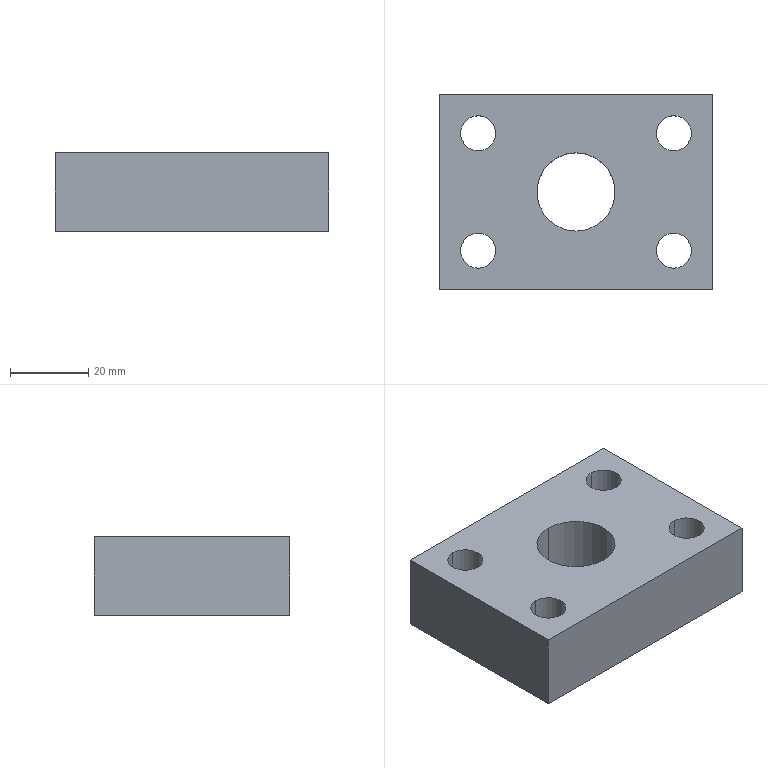Component | SolidWorks | UpperSideBeltXG-XG1-1_AdjustingNutXG1-1 | 1 solid | 16 faces | box 70 x 50 x 20 mm | volume 58627 mm3 | cylinder 10 | plane 6 | commonest cylinder face diameters 9 x8 20 x2
build123d program:
from build123d import *

# Parameters (mm, degrees)
SKETCH1_W                = 70
SKETCH1_H                = 50
BOSS_EXTRUDE1_DEPTH      = 10
F_9_0_9_DIAMETER_HOLE1_D = 9
M20_TAPPED_HOLE1_D       = 20


with BuildPart() as part:
    # Sketch1 → Boss-Extrude1 (new, symmetric)
    with BuildSketch(Plane(origin=(0, 0, 0), x_dir=(1, 0, 0), z_dir=(0, 1, 0))):
        Rectangle(SKETCH1_W, SKETCH1_H)
    extrude(amount=BOSS_EXTRUDE1_DEPTH, both=True)

    # 9.0 _9_ Diameter Hole1 (through all)
    with Locations(Plane(origin=(0, 10, 0), x_dir=(1, 0, 0), z_dir=(0, 1, 0))):
        with Locations((-25, 15), (-25, -15), (25, 15), (25, -15)):
            Hole(F_9_0_9_DIAMETER_HOLE1_D / 2)

    # M20 Tapped Hole1 (through all)
    with Locations(Plane(origin=(0, 10, 0), x_dir=(1, 0, 0), z_dir=(0, 1, 0))):
        with Locations((0, 0)):
            Hole(M20_TAPPED_HOLE1_D / 2)


solid = part.part

# Placed as in the assembly
solid = solid.moved(Location((-348.72, 470, 318), (90, 0, 0)))
STEP:
#1=CARTESIAN_POINT('',(-13.729,18.898,12.126));
#2=VERTEX_POINT('',#1);
#3=CARTESIAN_POINT('',(-13.729,18.11,12.126));
#4=VERTEX_POINT('',#3);
#5=CARTESIAN_POINT('',(-13.729,18.504,12.126));
#6=DIRECTION('',(0.,-0.,1.));
#7=DIRECTION('',(0.,-1.,0.));
#8=AXIS2_PLACEMENT_3D('',#5,#6,#7);
#9=CIRCLE('',#8,0.3937);
#10=EDGE_CURVE('',#2,#4,#9,.T.);
#11=ORIENTED_EDGE('',*,*,#10,.F.);
#12=CARTESIAN_POINT('',(-13.729,18.898,12.913));
#13=VERTEX_POINT('',#12);
#14=CARTESIAN_POINT('',(-13.729,18.898,12.913));
#15=DIRECTION('',(0.,-0.,1.));
#16=VECTOR('',#15,39.37);
#17=LINE('',#14,#16);
#18=EDGE_CURVE('',#2,#13,#17,.T.);
#19=ORIENTED_EDGE('',*,*,#18,.T.);
#20=CARTESIAN_POINT('',(-13.729,18.11,12.913));
#21=VERTEX_POINT('',#20);
#22=CARTESIAN_POINT('',(-13.729,18.504,12.913));
#23=DIRECTION('',(0.,-0.,1.));
#24=DIRECTION('',(0.,-1.,0.));
#25=AXIS2_PLACEMENT_3D('',#22,#23,#24);
#26=CIRCLE('',#25,0.3937);
#27=EDGE_CURVE('',#13,#21,#26,.T.);
#28=ORIENTED_EDGE('',*,*,#27,.T.);
#29=CARTESIAN_POINT('',(-13.729,18.11,12.913));
#30=DIRECTION('',(0.,-0.,1.));
#31=VECTOR('',#30,39.37);
#32=LINE('',#29,#31);
#33=EDGE_CURVE('',#4,#21,#32,.T.);
#34=ORIENTED_EDGE('',*,*,#33,.F.);
#35=EDGE_LOOP('',(#11,#19,#28,#34));
#36=FACE_OUTER_BOUND('',#35,.T.);
#37=CARTESIAN_POINT('',(-13.729,18.504,12.913));
#38=DIRECTION('',(0.,-0.,1.));
#39=DIRECTION('',(0.,-1.,0.));
#40=AXIS2_PLACEMENT_3D('',#37,#38,#39);
#41=CYLINDRICAL_SURFACE('',#40,0.3937);
#42=ADVANCED_FACE('',(#36),#41,.F.);
#43=CARTESIAN_POINT('',(-14.713,19.272,12.126));
#44=VERTEX_POINT('',#43);
#45=CARTESIAN_POINT('',(-14.713,18.917,12.126));
#46=VERTEX_POINT('',#45);
#47=CARTESIAN_POINT('',(-14.713,19.094,12.126));
#48=DIRECTION('',(0.,-0.,1.));
#49=DIRECTION('',(0.,-1.,0.));
#50=AXIS2_PLACEMENT_3D('',#47,#48,#49);
#51=CIRCLE('',#50,0.1772);
#52=EDGE_CURVE('',#44,#46,#51,.T.);
#53=ORIENTED_EDGE('',*,*,#52,.F.);
#54=CARTESIAN_POINT('',(-14.713,19.272,12.913));
#55=VERTEX_POINT('',#54);
#56=CARTESIAN_POINT('',(-14.713,19.272,12.913));
#57=DIRECTION('',(0.,-0.,1.));
#58=VECTOR('',#57,39.37);
#59=LINE('',#56,#58);
#60=EDGE_CURVE('',#44,#55,#59,.T.);
#61=ORIENTED_EDGE('',*,*,#60,.T.);
#62=CARTESIAN_POINT('',(-14.713,18.917,12.913));
#63=VERTEX_POINT('',#62);
#64=CARTESIAN_POINT('',(-14.713,19.094,12.913));
#65=DIRECTION('',(0.,-0.,1.));
#66=DIRECTION('',(0.,-1.,0.));
#67=AXIS2_PLACEMENT_3D('',#64,#65,#66);
#68=CIRCLE('',#67,0.1772);
#69=EDGE_CURVE('',#55,#63,#68,.T.);
#70=ORIENTED_EDGE('',*,*,#69,.T.);
#71=CARTESIAN_POINT('',(-14.713,18.917,12.913));
#72=DIRECTION('',(0.,-0.,1.));
#73=VECTOR('',#72,39.37);
#74=LINE('',#71,#73);
#75=EDGE_CURVE('',#46,#63,#74,.T.);
#76=ORIENTED_EDGE('',*,*,#75,.F.);
#77=EDGE_LOOP('',(#53,#61,#70,#76));
#78=FACE_OUTER_BOUND('',#77,.T.);
#79=CARTESIAN_POINT('',(-14.713,19.094,12.913));
#80=DIRECTION('',(0.,-0.,1.));
#81=DIRECTION('',(0.,-1.,0.));
#82=AXIS2_PLACEMENT_3D('',#79,#80,#81);
#83=CYLINDRICAL_SURFACE('',#82,0.1772);
#84=ADVANCED_FACE('',(#78),#83,.F.);
#85=CARTESIAN_POINT('',(-14.713,18.091,12.126));
#86=VERTEX_POINT('',#85);
#87=CARTESIAN_POINT('',(-14.713,17.736,12.126));
#88=VERTEX_POINT('',#87);
#89=CARTESIAN_POINT('',(-14.713,17.913,12.126));
#90=DIRECTION('',(0.,-0.,1.));
#91=DIRECTION('',(0.,-1.,0.));
#92=AXIS2_PLACEMENT_3D('',#89,#90,#91);
#93=CIRCLE('',#92,0.1772);
#94=EDGE_CURVE('',#86,#88,#93,.T.);
#95=ORIENTED_EDGE('',*,*,#94,.F.);
#96=CARTESIAN_POINT('',(-14.713,18.091,12.913));
#97=VERTEX_POINT('',#96);
#98=CARTESIAN_POINT('',(-14.713,18.091,12.913));
#99=DIRECTION('',(0.,-0.,1.));
#100=VECTOR('',#99,39.37);
#101=LINE('',#98,#100);
#102=EDGE_CURVE('',#86,#97,#101,.T.);
#103=ORIENTED_EDGE('',*,*,#102,.T.);
#104=CARTESIAN_POINT('',(-14.713,17.736,12.913));
#105=VERTEX_POINT('',#104);
#106=CARTESIAN_POINT('',(-14.713,17.913,12.913));
#107=DIRECTION('',(0.,-0.,1.));
#108=DIRECTION('',(0.,-1.,0.));
#109=AXIS2_PLACEMENT_3D('',#106,#107,#108);
#110=CIRCLE('',#109,0.1772);
#111=EDGE_CURVE('',#97,#105,#110,.T.);
#112=ORIENTED_EDGE('',*,*,#111,.T.);
#113=CARTESIAN_POINT('',(-14.713,17.736,12.913));
#114=DIRECTION('',(0.,-0.,1.));
#115=VECTOR('',#114,39.37);
#116=LINE('',#113,#115);
#117=EDGE_CURVE('',#88,#105,#116,.T.);
#118=ORIENTED_EDGE('',*,*,#117,.F.);
#119=EDGE_LOOP('',(#95,#103,#112,#118));
#120=FACE_OUTER_BOUND('',#119,.T.);
#121=CARTESIAN_POINT('',(-14.713,17.913,12.913));
#122=DIRECTION('',(0.,-0.,1.));
#123=DIRECTION('',(0.,-1.,0.));
#124=AXIS2_PLACEMENT_3D('',#121,#122,#123);
#125=CYLINDRICAL_SURFACE('',#124,0.1772);
#126=ADVANCED_FACE('',(#120),#125,.F.);
#127=CARTESIAN_POINT('',(-12.745,19.272,12.126));
#128=VERTEX_POINT('',#127);
#129=CARTESIAN_POINT('',(-12.745,18.917,12.126));
#130=VERTEX_POINT('',#129);
#131=CARTESIAN_POINT('',(-12.745,19.094,12.126));
#132=DIRECTION('',(0.,-0.,1.));
#133=DIRECTION('',(0.,-1.,0.));
#134=AXIS2_PLACEMENT_3D('',#131,#132,#133);
#135=CIRCLE('',#134,0.1772);
#136=EDGE_CURVE('',#128,#130,#135,.T.);
#137=ORIENTED_EDGE('',*,*,#136,.F.);
#138=CARTESIAN_POINT('',(-12.745,19.272,12.913));
#139=VERTEX_POINT('',#138);
#140=CARTESIAN_POINT('',(-12.745,19.272,12.913));
#141=DIRECTION('',(0.,-0.,1.));
#142=VECTOR('',#141,39.37);
#143=LINE('',#140,#142);
#144=EDGE_CURVE('',#128,#139,#143,.T.);
#145=ORIENTED_EDGE('',*,*,#144,.T.);
#146=CARTESIAN_POINT('',(-12.745,18.917,12.913));
#147=VERTEX_POINT('',#146);
#148=CARTESIAN_POINT('',(-12.745,19.094,12.913));
#149=DIRECTION('',(0.,-0.,1.));
#150=DIRECTION('',(0.,-1.,0.));
#151=AXIS2_PLACEMENT_3D('',#148,#149,#150);
#152=CIRCLE('',#151,0.1772);
#153=EDGE_CURVE('',#139,#147,#152,.T.);
#154=ORIENTED_EDGE('',*,*,#153,.T.);
#155=CARTESIAN_POINT('',(-12.745,18.917,12.913));
#156=DIRECTION('',(0.,-0.,1.));
#157=VECTOR('',#156,39.37);
#158=LINE('',#155,#157);
#159=EDGE_CURVE('',#130,#147,#158,.T.);
#160=ORIENTED_EDGE('',*,*,#159,.F.);
#161=EDGE_LOOP('',(#137,#145,#154,#160));
#162=FACE_OUTER_BOUND('',#161,.T.);
#163=CARTESIAN_POINT('',(-12.745,19.094,12.913));
#164=DIRECTION('',(0.,-0.,1.));
#165=DIRECTION('',(0.,-1.,0.));
#166=AXIS2_PLACEMENT_3D('',#163,#164,#165);
#167=CYLINDRICAL_SURFACE('',#166,0.1772);
#168=ADVANCED_FACE('',(#162),#167,.F.);
#169=CARTESIAN_POINT('',(-12.745,18.091,12.126));
#170=VERTEX_POINT('',#169);
#171=CARTESIAN_POINT('',(-12.745,17.736,12.126));
#172=VERTEX_POINT('',#171);
#173=CARTESIAN_POINT('',(-12.745,17.913,12.126));
#174=DIRECTION('',(0.,-0.,1.));
#175=DIRECTION('',(0.,-1.,0.));
#176=AXIS2_PLACEMENT_3D('',#173,#174,#175);
#177=CIRCLE('',#176,0.1772);
#178=EDGE_CURVE('',#170,#172,#177,.T.);
#179=ORIENTED_EDGE('',*,*,#178,.F.);
#180=CARTESIAN_POINT('',(-12.745,18.091,12.913));
#181=VERTEX_POINT('',#180);
#182=CARTESIAN_POINT('',(-12.745,18.091,12.913));
#183=DIRECTION('',(0.,-0.,1.));
#184=VECTOR('',#183,39.37);
#185=LINE('',#182,#184);
#186=EDGE_CURVE('',#170,#181,#185,.T.);
#187=ORIENTED_EDGE('',*,*,#186,.T.);
#188=CARTESIAN_POINT('',(-12.745,17.736,12.913));
#189=VERTEX_POINT('',#188);
#190=CARTESIAN_POINT('',(-12.745,17.913,12.913));
#191=DIRECTION('',(0.,-0.,1.));
#192=DIRECTION('',(0.,-1.,0.));
#193=AXIS2_PLACEMENT_3D('',#190,#191,#192);
#194=CIRCLE('',#193,0.1772);
#195=EDGE_CURVE('',#181,#189,#194,.T.);
#196=ORIENTED_EDGE('',*,*,#195,.T.);
#197=CARTESIAN_POINT('',(-12.745,17.736,12.913));
#198=DIRECTION('',(0.,-0.,1.));
#199=VECTOR('',#198,39.37);
#200=LINE('',#197,#199);
#201=EDGE_CURVE('',#172,#189,#200,.T.);
#202=ORIENTED_EDGE('',*,*,#201,.F.);
#203=EDGE_LOOP('',(#179,#187,#196,#202));
#204=FACE_OUTER_BOUND('',#203,.T.);
#205=CARTESIAN_POINT('',(-12.745,17.913,12.913));
#206=DIRECTION('',(0.,-0.,1.));
#207=DIRECTION('',(0.,-1.,0.));
#208=AXIS2_PLACEMENT_3D('',#205,#206,#207);
#209=CYLINDRICAL_SURFACE('',#208,0.1772);
#210=ADVANCED_FACE('',(#204),#209,.F.);
#211=CARTESIAN_POINT('',(-15.107,19.488,12.126));
#212=VERTEX_POINT('',#211);
#213=CARTESIAN_POINT('',(-15.107,17.52,12.126));
#214=VERTEX_POINT('',#213);
#215=CARTESIAN_POINT('',(-15.107,17.52,12.126));
#216=DIRECTION('',(-0.,-1.,-0.));
#217=VECTOR('',#216,39.37);
#218=LINE('',#215,#217);
#219=EDGE_CURVE('',#212,#214,#218,.T.);
#220=ORIENTED_EDGE('',*,*,#219,.T.);
#221=CARTESIAN_POINT('',(-15.107,17.52,12.913));
#222=VERTEX_POINT('',#221);
#223=CARTESIAN_POINT('',(-15.107,17.52,12.913));
#224=DIRECTION('',(-0.,0.,-1.));
#225=VECTOR('',#224,39.37);
#226=LINE('',#223,#225);
#227=EDGE_CURVE('',#222,#214,#226,.T.);
#228=ORIENTED_EDGE('',*,*,#227,.F.);
#229=CARTESIAN_POINT('',(-15.107,19.488,12.913));
#230=VERTEX_POINT('',#229);
#231=CARTESIAN_POINT('',(-15.107,17.52,12.913));
#232=DIRECTION('',(-0.,-1.,-0.));
#233=VECTOR('',#232,39.37);
#234=LINE('',#231,#233);
#235=EDGE_CURVE('',#230,#222,#234,.T.);
#236=ORIENTED_EDGE('',*,*,#235,.F.);
#237=CARTESIAN_POINT('',(-15.107,19.488,12.913));
#238=DIRECTION('',(-0.,0.,-1.));
#239=VECTOR('',#238,39.37);
#240=LINE('',#237,#239);
#241=EDGE_CURVE('',#230,#212,#240,.T.);
#242=ORIENTED_EDGE('',*,*,#241,.T.);
#243=EDGE_LOOP('',(#220,#228,#236,#242));
#244=FACE_OUTER_BOUND('',#243,.T.);
#245=CARTESIAN_POINT('',(-15.107,17.52,12.913));
#246=DIRECTION('',(1.,-0.,-0.));
#247=DIRECTION('',(0.,1.,0.));
#248=AXIS2_PLACEMENT_3D('',#245,#246,#247);
#249=PLANE('',#248);
#250=ADVANCED_FACE('',(#244),#249,.F.);
#251=CARTESIAN_POINT('',(-12.351,17.52,12.126));
#252=VERTEX_POINT('',#251);
#253=CARTESIAN_POINT('',(-12.351,17.52,12.126));
#254=DIRECTION('',(1.,-0.,-0.));
#255=VECTOR('',#254,39.37);
#256=LINE('',#253,#255);
#257=EDGE_CURVE('',#214,#252,#256,.T.);
#258=ORIENTED_EDGE('',*,*,#257,.T.);
#259=CARTESIAN_POINT('',(-12.351,17.52,12.913));
#260=VERTEX_POINT('',#259);
#261=CARTESIAN_POINT('',(-12.351,17.52,12.913));
#262=DIRECTION('',(-0.,0.,-1.));
#263=VECTOR('',#262,39.37);
#264=LINE('',#261,#263);
#265=EDGE_CURVE('',#260,#252,#264,.T.);
#266=ORIENTED_EDGE('',*,*,#265,.F.);
#267=CARTESIAN_POINT('',(-12.351,17.52,12.913));
#268=DIRECTION('',(1.,-0.,-0.));
#269=VECTOR('',#268,39.37);
#270=LINE('',#267,#269);
#271=EDGE_CURVE('',#222,#260,#270,.T.);
#272=ORIENTED_EDGE('',*,*,#271,.F.);
#273=ORIENTED_EDGE('',*,*,#227,.T.);
#274=EDGE_LOOP('',(#258,#266,#272,#273));
#275=FACE_OUTER_BOUND('',#274,.T.);
#276=CARTESIAN_POINT('',(-12.351,17.52,12.913));
#277=DIRECTION('',(0.,1.,0.));
#278=DIRECTION('',(-1.,0.,0.));
#279=AXIS2_PLACEMENT_3D('',#276,#277,#278);
#280=PLANE('',#279);
#281=ADVANCED_FACE('',(#275),#280,.F.);
#282=CARTESIAN_POINT('',(-12.351,19.488,12.126));
#283=VERTEX_POINT('',#282);
#284=CARTESIAN_POINT('',(-12.351,17.52,12.126));
#285=DIRECTION('',(0.,1.,0.));
#286=VECTOR('',#285,39.37);
#287=LINE('',#284,#286);
#288=EDGE_CURVE('',#252,#283,#287,.T.);
#289=ORIENTED_EDGE('',*,*,#288,.T.);
#290=CARTESIAN_POINT('',(-12.351,19.488,12.913));
#291=VERTEX_POINT('',#290);
#292=CARTESIAN_POINT('',(-12.351,19.488,12.913));
#293=DIRECTION('',(-0.,0.,-1.));
#294=VECTOR('',#293,39.37);
#295=LINE('',#292,#294);
#296=EDGE_CURVE('',#291,#283,#295,.T.);
#297=ORIENTED_EDGE('',*,*,#296,.F.);
#298=CARTESIAN_POINT('',(-12.351,17.52,12.913));
#299=DIRECTION('',(0.,1.,0.));
#300=VECTOR('',#299,39.37);
#301=LINE('',#298,#300);
#302=EDGE_CURVE('',#260,#291,#301,.T.);
#303=ORIENTED_EDGE('',*,*,#302,.F.);
#304=ORIENTED_EDGE('',*,*,#265,.T.);
#305=EDGE_LOOP('',(#289,#297,#303,#304));
#306=FACE_OUTER_BOUND('',#305,.T.);
#307=CARTESIAN_POINT('',(-12.351,17.52,12.913));
#308=DIRECTION('',(-1.,0.,0.));
#309=DIRECTION('',(-0.,-1.,-0.));
#310=AXIS2_PLACEMENT_3D('',#307,#308,#309);
#311=PLANE('',#310);
#312=ADVANCED_FACE('',(#306),#311,.F.);
#313=CARTESIAN_POINT('',(-12.351,19.488,12.126));
#314=DIRECTION('',(-1.,0.,0.));
#315=VECTOR('',#314,39.37);
#316=LINE('',#313,#315);
#317=EDGE_CURVE('',#283,#212,#316,.T.);
#318=ORIENTED_EDGE('',*,*,#317,.T.);
#319=ORIENTED_EDGE('',*,*,#241,.F.);
#320=CARTESIAN_POINT('',(-12.351,19.488,12.913));
#321=DIRECTION('',(-1.,0.,0.));
#322=VECTOR('',#321,39.37);
#323=LINE('',#320,#322);
#324=EDGE_CURVE('',#291,#230,#323,.T.);
#325=ORIENTED_EDGE('',*,*,#324,.F.);
#326=ORIENTED_EDGE('',*,*,#296,.T.);
#327=EDGE_LOOP('',(#318,#319,#325,#326));
#328=FACE_OUTER_BOUND('',#327,.T.);
#329=CARTESIAN_POINT('',(-12.351,19.488,12.913));
#330=DIRECTION('',(-0.,-1.,-0.));
#331=DIRECTION('',(1.,-0.,-0.));
#332=AXIS2_PLACEMENT_3D('',#329,#330,#331);
#333=PLANE('',#332);
#334=ADVANCED_FACE('',(#328),#333,.F.);
#335=CARTESIAN_POINT('',(-13.729,18.504,12.913));
#336=DIRECTION('',(0.,-0.,1.));
#337=DIRECTION('',(0.,-1.,0.));
#338=AXIS2_PLACEMENT_3D('',#335,#336,#337);
#339=CIRCLE('',#338,0.3937);
#340=EDGE_CURVE('',#21,#13,#339,.T.);
#341=ORIENTED_EDGE('',*,*,#340,.F.);
#342=ORIENTED_EDGE('',*,*,#27,.F.);
#343=EDGE_LOOP('',(#341,#342));
#344=FACE_BOUND('',#343,.T.);
#345=CARTESIAN_POINT('',(-14.713,19.094,12.913));
#346=DIRECTION('',(0.,-0.,1.));
#347=DIRECTION('',(0.,-1.,0.));
#348=AXIS2_PLACEMENT_3D('',#345,#346,#347);
#349=CIRCLE('',#348,0.1772);
#350=EDGE_CURVE('',#63,#55,#349,.T.);
#351=ORIENTED_EDGE('',*,*,#350,.F.);
#352=ORIENTED_EDGE('',*,*,#69,.F.);
#353=EDGE_LOOP('',(#351,#352));
#354=FACE_BOUND('',#353,.T.);
#355=CARTESIAN_POINT('',(-14.713,17.913,12.913));
#356=DIRECTION('',(0.,-0.,1.));
#357=DIRECTION('',(0.,-1.,0.));
#358=AXIS2_PLACEMENT_3D('',#355,#356,#357);
#359=CIRCLE('',#358,0.1772);
#360=EDGE_CURVE('',#105,#97,#359,.T.);
#361=ORIENTED_EDGE('',*,*,#360,.F.);
#362=ORIENTED_EDGE('',*,*,#111,.F.);
#363=EDGE_LOOP('',(#361,#362));
#364=FACE_BOUND('',#363,.T.);
#365=CARTESIAN_POINT('',(-12.745,19.094,12.913));
#366=DIRECTION('',(0.,-0.,1.));
#367=DIRECTION('',(0.,-1.,0.));
#368=AXIS2_PLACEMENT_3D('',#365,#366,#367);
#369=CIRCLE('',#368,0.1772);
#370=EDGE_CURVE('',#147,#139,#369,.T.);
#371=ORIENTED_EDGE('',*,*,#370,.F.);
#372=ORIENTED_EDGE('',*,*,#153,.F.);
#373=EDGE_LOOP('',(#371,#372));
#374=FACE_BOUND('',#373,.T.);
#375=CARTESIAN_POINT('',(-12.745,17.913,12.913));
#376=DIRECTION('',(0.,-0.,1.));
#377=DIRECTION('',(0.,-1.,0.));
#378=AXIS2_PLACEMENT_3D('',#375,#376,#377);
#379=CIRCLE('',#378,0.1772);
#380=EDGE_CURVE('',#189,#181,#379,.T.);
#381=ORIENTED_EDGE('',*,*,#380,.F.);
#382=ORIENTED_EDGE('',*,*,#195,.F.);
#383=EDGE_LOOP('',(#381,#382));
#384=FACE_BOUND('',#383,.T.);
#385=ORIENTED_EDGE('',*,*,#235,.T.);
#386=ORIENTED_EDGE('',*,*,#271,.T.);
#387=ORIENTED_EDGE('',*,*,#302,.T.);
#388=ORIENTED_EDGE('',*,*,#324,.T.);
#389=EDGE_LOOP('',(#385,#386,#387,#388));
#390=FACE_OUTER_BOUND('',#389,.T.);
#391=CARTESIAN_POINT('',(-13.729,18.504,12.913));
#392=DIRECTION('',(0.,-0.,1.));
#393=DIRECTION('',(-0.,-1.,-0.));
#394=AXIS2_PLACEMENT_3D('',#391,#392,#393);
#395=PLANE('',#394);
#396=ADVANCED_FACE('',(#344,#354,#364,#374,#384,#390),#395,.T.);
#397=CARTESIAN_POINT('',(-13.729,18.504,12.126));
#398=DIRECTION('',(0.,-0.,1.));
#399=DIRECTION('',(0.,-1.,0.));
#400=AXIS2_PLACEMENT_3D('',#397,#398,#399);
#401=CIRCLE('',#400,0.3937);
#402=EDGE_CURVE('',#4,#2,#401,.T.);
#403=ORIENTED_EDGE('',*,*,#402,.T.);
#404=ORIENTED_EDGE('',*,*,#10,.T.);
#405=EDGE_LOOP('',(#403,#404));
#406=FACE_BOUND('',#405,.T.);
#407=CARTESIAN_POINT('',(-14.713,19.094,12.126));
#408=DIRECTION('',(0.,-0.,1.));
#409=DIRECTION('',(0.,-1.,0.));
#410=AXIS2_PLACEMENT_3D('',#407,#408,#409);
#411=CIRCLE('',#410,0.1772);
#412=EDGE_CURVE('',#46,#44,#411,.T.);
#413=ORIENTED_EDGE('',*,*,#412,.T.);
#414=ORIENTED_EDGE('',*,*,#52,.T.);
#415=EDGE_LOOP('',(#413,#414));
#416=FACE_BOUND('',#415,.T.);
#417=CARTESIAN_POINT('',(-14.713,17.913,12.126));
#418=DIRECTION('',(0.,-0.,1.));
#419=DIRECTION('',(0.,-1.,0.));
#420=AXIS2_PLACEMENT_3D('',#417,#418,#419);
#421=CIRCLE('',#420,0.1772);
#422=EDGE_CURVE('',#88,#86,#421,.T.);
#423=ORIENTED_EDGE('',*,*,#422,.T.);
#424=ORIENTED_EDGE('',*,*,#94,.T.);
#425=EDGE_LOOP('',(#423,#424));
#426=FACE_BOUND('',#425,.T.);
#427=CARTESIAN_POINT('',(-12.745,19.094,12.126));
#428=DIRECTION('',(0.,-0.,1.));
#429=DIRECTION('',(0.,-1.,0.));
#430=AXIS2_PLACEMENT_3D('',#427,#428,#429);
#431=CIRCLE('',#430,0.1772);
#432=EDGE_CURVE('',#130,#128,#431,.T.);
#433=ORIENTED_EDGE('',*,*,#432,.T.);
#434=ORIENTED_EDGE('',*,*,#136,.T.);
#435=EDGE_LOOP('',(#433,#434));
#436=FACE_BOUND('',#435,.T.);
#437=CARTESIAN_POINT('',(-12.745,17.913,12.126));
#438=DIRECTION('',(0.,-0.,1.));
#439=DIRECTION('',(0.,-1.,0.));
#440=AXIS2_PLACEMENT_3D('',#437,#438,#439);
#441=CIRCLE('',#440,0.1772);
#442=EDGE_CURVE('',#172,#170,#441,.T.);
#443=ORIENTED_EDGE('',*,*,#442,.T.);
#444=ORIENTED_EDGE('',*,*,#178,.T.);
#445=EDGE_LOOP('',(#443,#444));
#446=FACE_BOUND('',#445,.T.);
#447=ORIENTED_EDGE('',*,*,#219,.F.);
#448=ORIENTED_EDGE('',*,*,#317,.F.);
#449=ORIENTED_EDGE('',*,*,#288,.F.);
#450=ORIENTED_EDGE('',*,*,#257,.F.);
#451=EDGE_LOOP('',(#447,#448,#449,#450));
#452=FACE_OUTER_BOUND('',#451,.T.);
#453=CARTESIAN_POINT('',(-13.729,18.504,12.126));
#454=DIRECTION('',(0.,-0.,1.));
#455=DIRECTION('',(-0.,-1.,-0.));
#456=AXIS2_PLACEMENT_3D('',#453,#454,#455);
#457=PLANE('',#456);
#458=ADVANCED_FACE('',(#406,#416,#426,#436,#446,#452),#457,.F.);
#459=ORIENTED_EDGE('',*,*,#186,.F.);
#460=ORIENTED_EDGE('',*,*,#442,.F.);
#461=ORIENTED_EDGE('',*,*,#201,.T.);
#462=ORIENTED_EDGE('',*,*,#380,.T.);
#463=EDGE_LOOP('',(#459,#460,#461,#462));
#464=FACE_OUTER_BOUND('',#463,.T.);
#465=CARTESIAN_POINT('',(-12.745,17.913,12.913));
#466=DIRECTION('',(0.,-0.,1.));
#467=DIRECTION('',(0.,-1.,0.));
#468=AXIS2_PLACEMENT_3D('',#465,#466,#467);
#469=CYLINDRICAL_SURFACE('',#468,0.1772);
#470=ADVANCED_FACE('',(#464),#469,.F.);
#471=ORIENTED_EDGE('',*,*,#144,.F.);
#472=ORIENTED_EDGE('',*,*,#432,.F.);
#473=ORIENTED_EDGE('',*,*,#159,.T.);
#474=ORIENTED_EDGE('',*,*,#370,.T.);
#475=EDGE_LOOP('',(#471,#472,#473,#474));
#476=FACE_OUTER_BOUND('',#475,.T.);
#477=CARTESIAN_POINT('',(-12.745,19.094,12.913));
#478=DIRECTION('',(0.,-0.,1.));
#479=DIRECTION('',(0.,-1.,0.));
#480=AXIS2_PLACEMENT_3D('',#477,#478,#479);
#481=CYLINDRICAL_SURFACE('',#480,0.1772);
#482=ADVANCED_FACE('',(#476),#481,.F.);
#483=ORIENTED_EDGE('',*,*,#102,.F.);
#484=ORIENTED_EDGE('',*,*,#422,.F.);
#485=ORIENTED_EDGE('',*,*,#117,.T.);
#486=ORIENTED_EDGE('',*,*,#360,.T.);
#487=EDGE_LOOP('',(#483,#484,#485,#486));
#488=FACE_OUTER_BOUND('',#487,.T.);
#489=CARTESIAN_POINT('',(-14.713,17.913,12.913));
#490=DIRECTION('',(0.,-0.,1.));
#491=DIRECTION('',(0.,-1.,0.));
#492=AXIS2_PLACEMENT_3D('',#489,#490,#491);
#493=CYLINDRICAL_SURFACE('',#492,0.1772);
#494=ADVANCED_FACE('',(#488),#493,.F.);
#495=ORIENTED_EDGE('',*,*,#60,.F.);
#496=ORIENTED_EDGE('',*,*,#412,.F.);
#497=ORIENTED_EDGE('',*,*,#75,.T.);
#498=ORIENTED_EDGE('',*,*,#350,.T.);
#499=EDGE_LOOP('',(#495,#496,#497,#498));
#500=FACE_OUTER_BOUND('',#499,.T.);
#501=CARTESIAN_POINT('',(-14.713,19.094,12.913));
#502=DIRECTION('',(0.,-0.,1.));
#503=DIRECTION('',(0.,-1.,0.));
#504=AXIS2_PLACEMENT_3D('',#501,#502,#503);
#505=CYLINDRICAL_SURFACE('',#504,0.1772);
#506=ADVANCED_FACE('',(#500),#505,.F.);
#507=ORIENTED_EDGE('',*,*,#18,.F.);
#508=ORIENTED_EDGE('',*,*,#402,.F.);
#509=ORIENTED_EDGE('',*,*,#33,.T.);
#510=ORIENTED_EDGE('',*,*,#340,.T.);
#511=EDGE_LOOP('',(#507,#508,#509,#510));
#512=FACE_OUTER_BOUND('',#511,.T.);
#513=CARTESIAN_POINT('',(-13.729,18.504,12.913));
#514=DIRECTION('',(0.,-0.,1.));
#515=DIRECTION('',(0.,-1.,0.));
#516=AXIS2_PLACEMENT_3D('',#513,#514,#515);
#517=CYLINDRICAL_SURFACE('',#516,0.3937);
#518=ADVANCED_FACE('',(#512),#517,.F.);
#519=CLOSED_SHELL('',(#42,#84,#126,#168,#210,#250,#281,#312,#334,#396,#458,#470,#482,#494,#506,#518));
#520=MANIFOLD_SOLID_BREP('',#519);
#521=CARTESIAN_POINT('',(0.,0.,0.));
#522=DIRECTION('',(0.,0.,1.));
#523=DIRECTION('',(1.,0.,0.));
#524=AXIS2_PLACEMENT_3D('',#521,#522,#523);
#525=(LENGTH_UNIT()NAMED_UNIT(*)SI_UNIT($,.METRE.));
#526=LENGTH_MEASURE_WITH_UNIT(LENGTH_MEASURE(0.0254),#525);
#527=DIMENSIONAL_EXPONENTS(1.,0.,0.,0.,0.,0.,0.);
#528=(CONVERSION_BASED_UNIT('',#526)LENGTH_UNIT()NAMED_UNIT(#527));
#529=UNCERTAINTY_MEASURE_WITH_UNIT(LENGTH_MEASURE(0.00001),#528,'','');
#530=(NAMED_UNIT(*)PLANE_ANGLE_UNIT()SI_UNIT($,.RADIAN.));
#531=(NAMED_UNIT(*)SI_UNIT($,.STERADIAN.)SOLID_ANGLE_UNIT());
#532=(GEOMETRIC_REPRESENTATION_CONTEXT(3)GLOBAL_UNCERTAINTY_ASSIGNED_CONTEXT((#529))GLOBAL_UNIT_ASSIGNED_CONTEXT((#528,#530,#531))REPRESENTATION_CONTEXT('',''));
#533=ADVANCED_BREP_SHAPE_REPRESENTATION('',(#520,#524),#532);
#534=COLOUR_RGB('',0.7922,0.8196,0.9333);
#535=FILL_AREA_STYLE_COLOUR('',#534);
#536=FILL_AREA_STYLE('',(#535));
#537=SURFACE_STYLE_FILL_AREA(#536);
#538=SURFACE_SIDE_STYLE('',(#537));
#539=SURFACE_STYLE_USAGE(.BOTH.,#538);
#540=PRESENTATION_STYLE_ASSIGNMENT((#539));
#541=STYLED_ITEM('',(#540),#520);
#542=PRESENTATION_LAYER_ASSIGNMENT('','',(#541));
#543=(LENGTH_UNIT()NAMED_UNIT(*)SI_UNIT($,.METRE.));
#544=LENGTH_MEASURE_WITH_UNIT(LENGTH_MEASURE(0.0254),#543);
#545=DIMENSIONAL_EXPONENTS(1.,0.,0.,0.,0.,0.,0.);
#546=(CONVERSION_BASED_UNIT('',#544)LENGTH_UNIT()NAMED_UNIT(#545));
#547=UNCERTAINTY_MEASURE_WITH_UNIT(LENGTH_MEASURE(0.00001),#546,'','');
#548=(NAMED_UNIT(*)PLANE_ANGLE_UNIT()SI_UNIT($,.RADIAN.));
#549=(NAMED_UNIT(*)SI_UNIT($,.STERADIAN.)SOLID_ANGLE_UNIT());
#550=(GEOMETRIC_REPRESENTATION_CONTEXT(3)GLOBAL_UNCERTAINTY_ASSIGNED_CONTEXT((#547))GLOBAL_UNIT_ASSIGNED_CONTEXT((#546,#548,#549))REPRESENTATION_CONTEXT('',''));
#551=MECHANICAL_DESIGN_GEOMETRIC_PRESENTATION_REPRESENTATION('',(#541),#550);